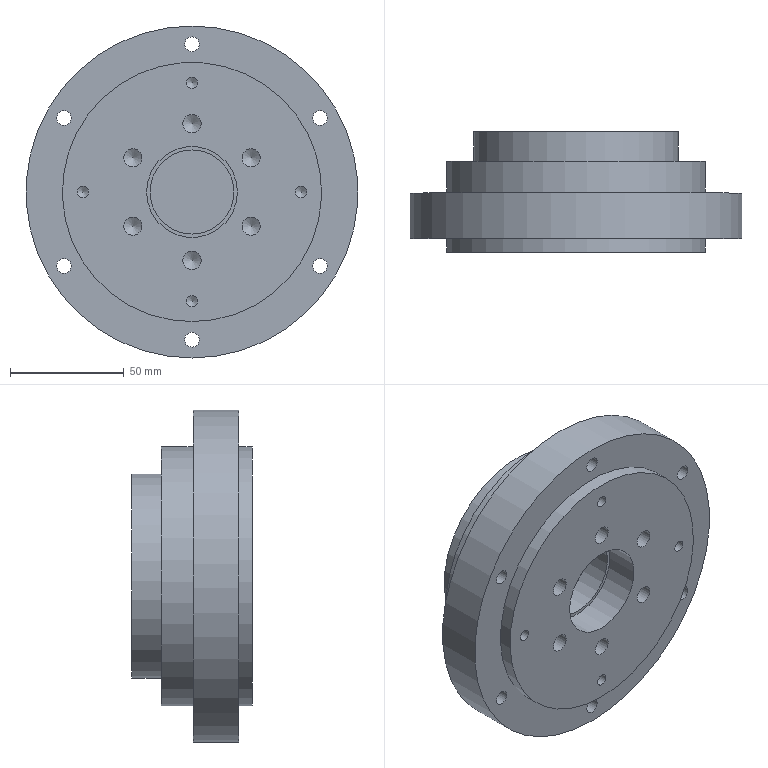Component | NX | COVER | 1 solid | 39 faces | volume 572810 mm3 | cylinder 22 | cone 10 | plane 7 | commonest cylinder face diameters 8 x6 6.5 x6 5 x4 114 x2 146 x1 90 x1 40 x1 37 x1